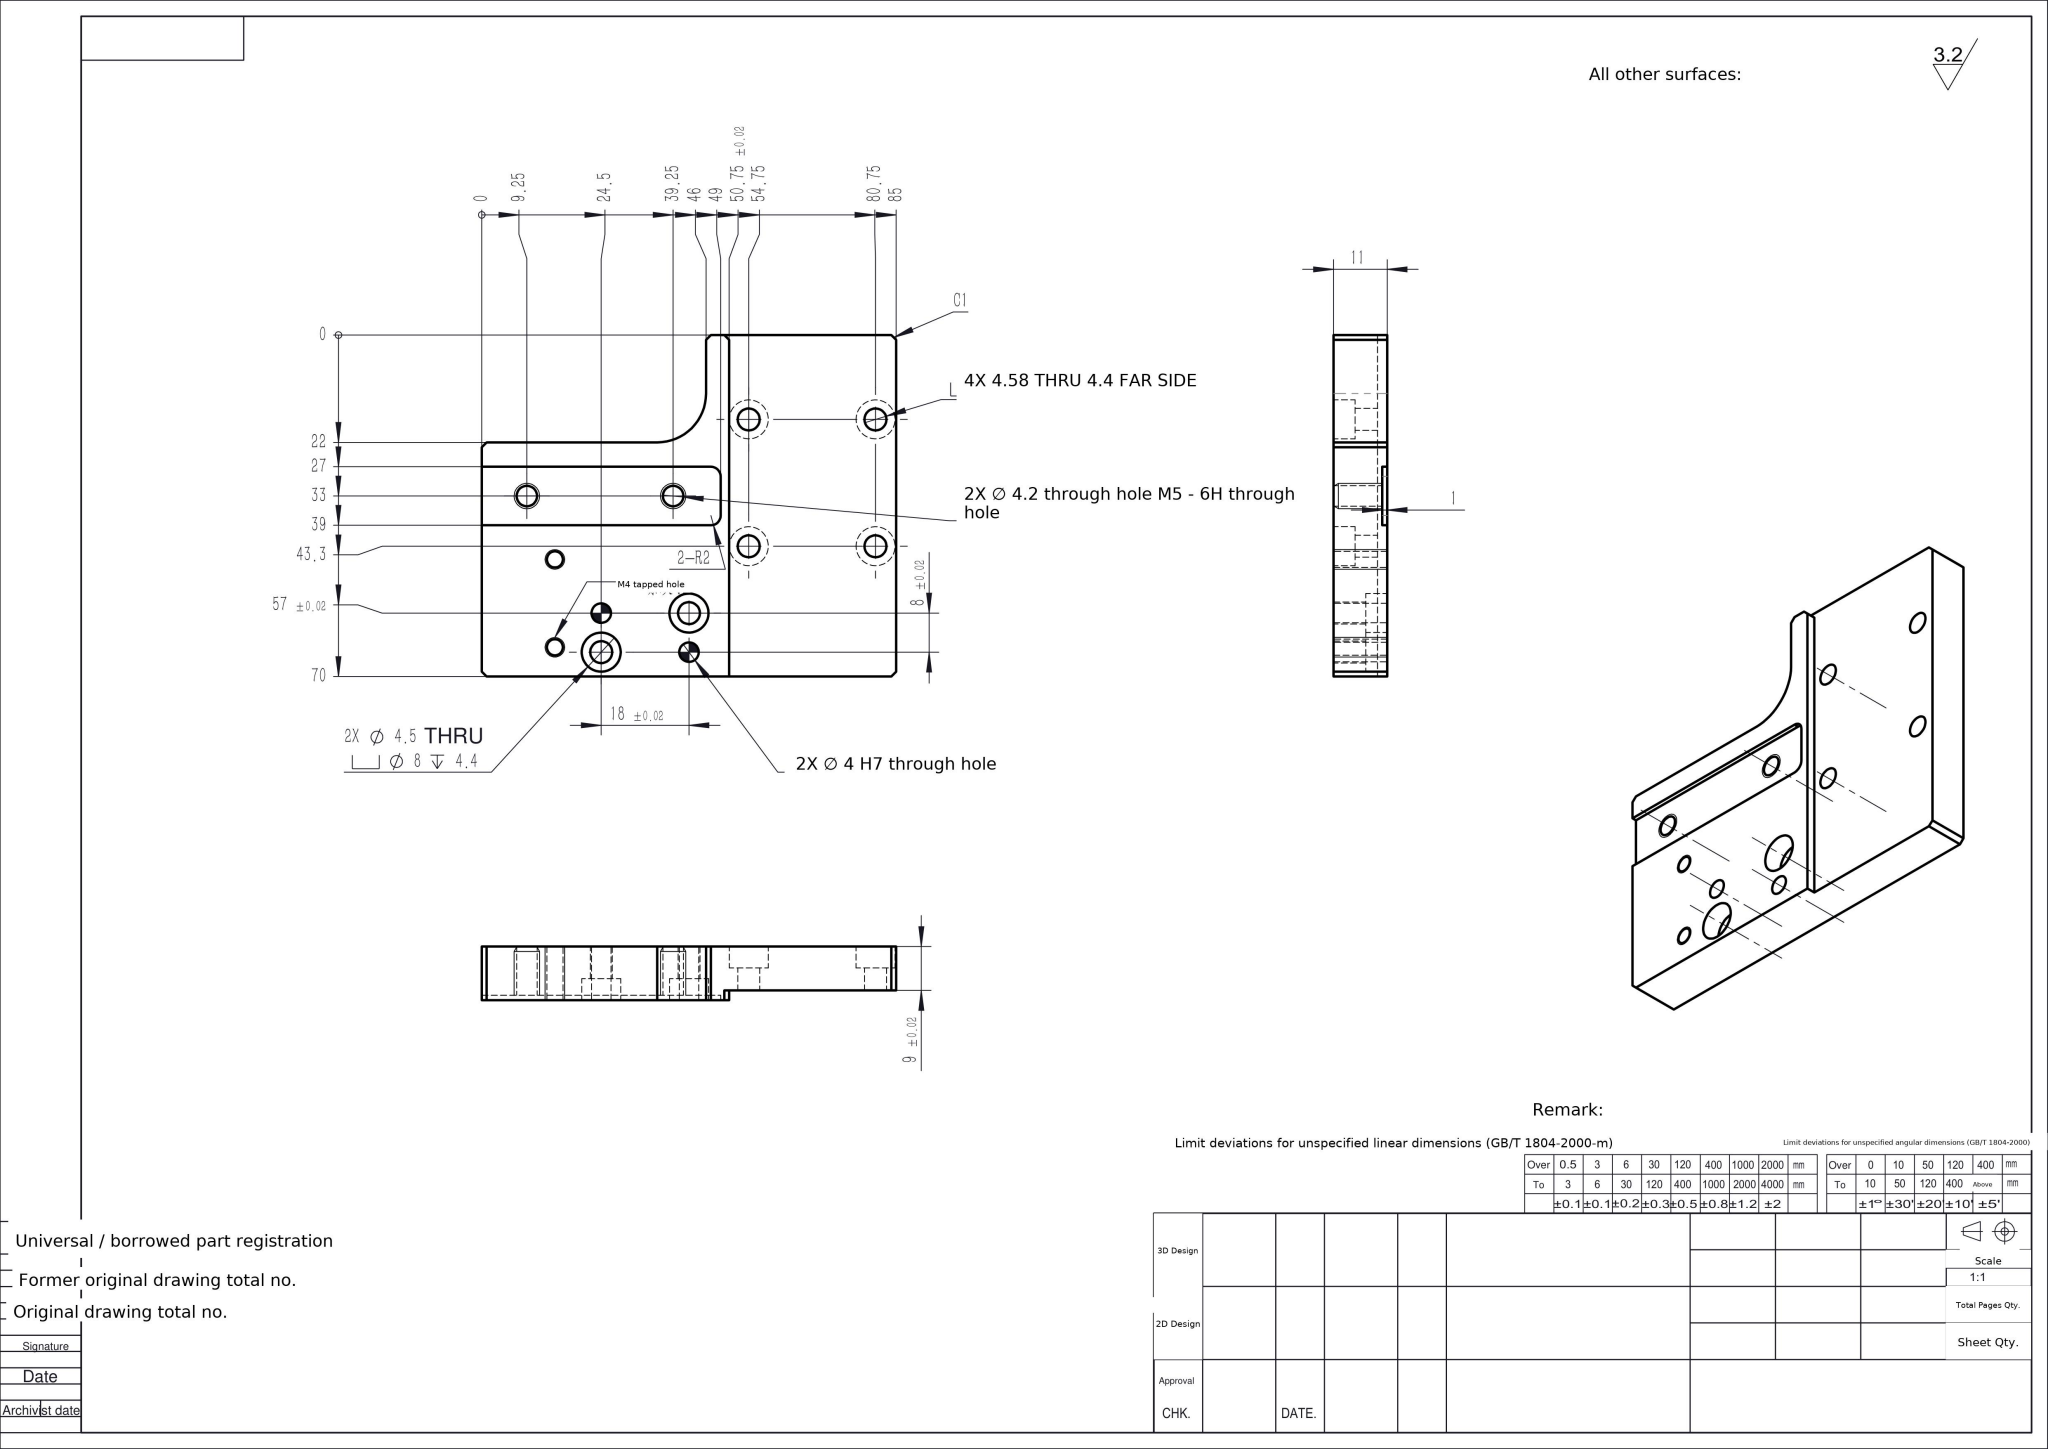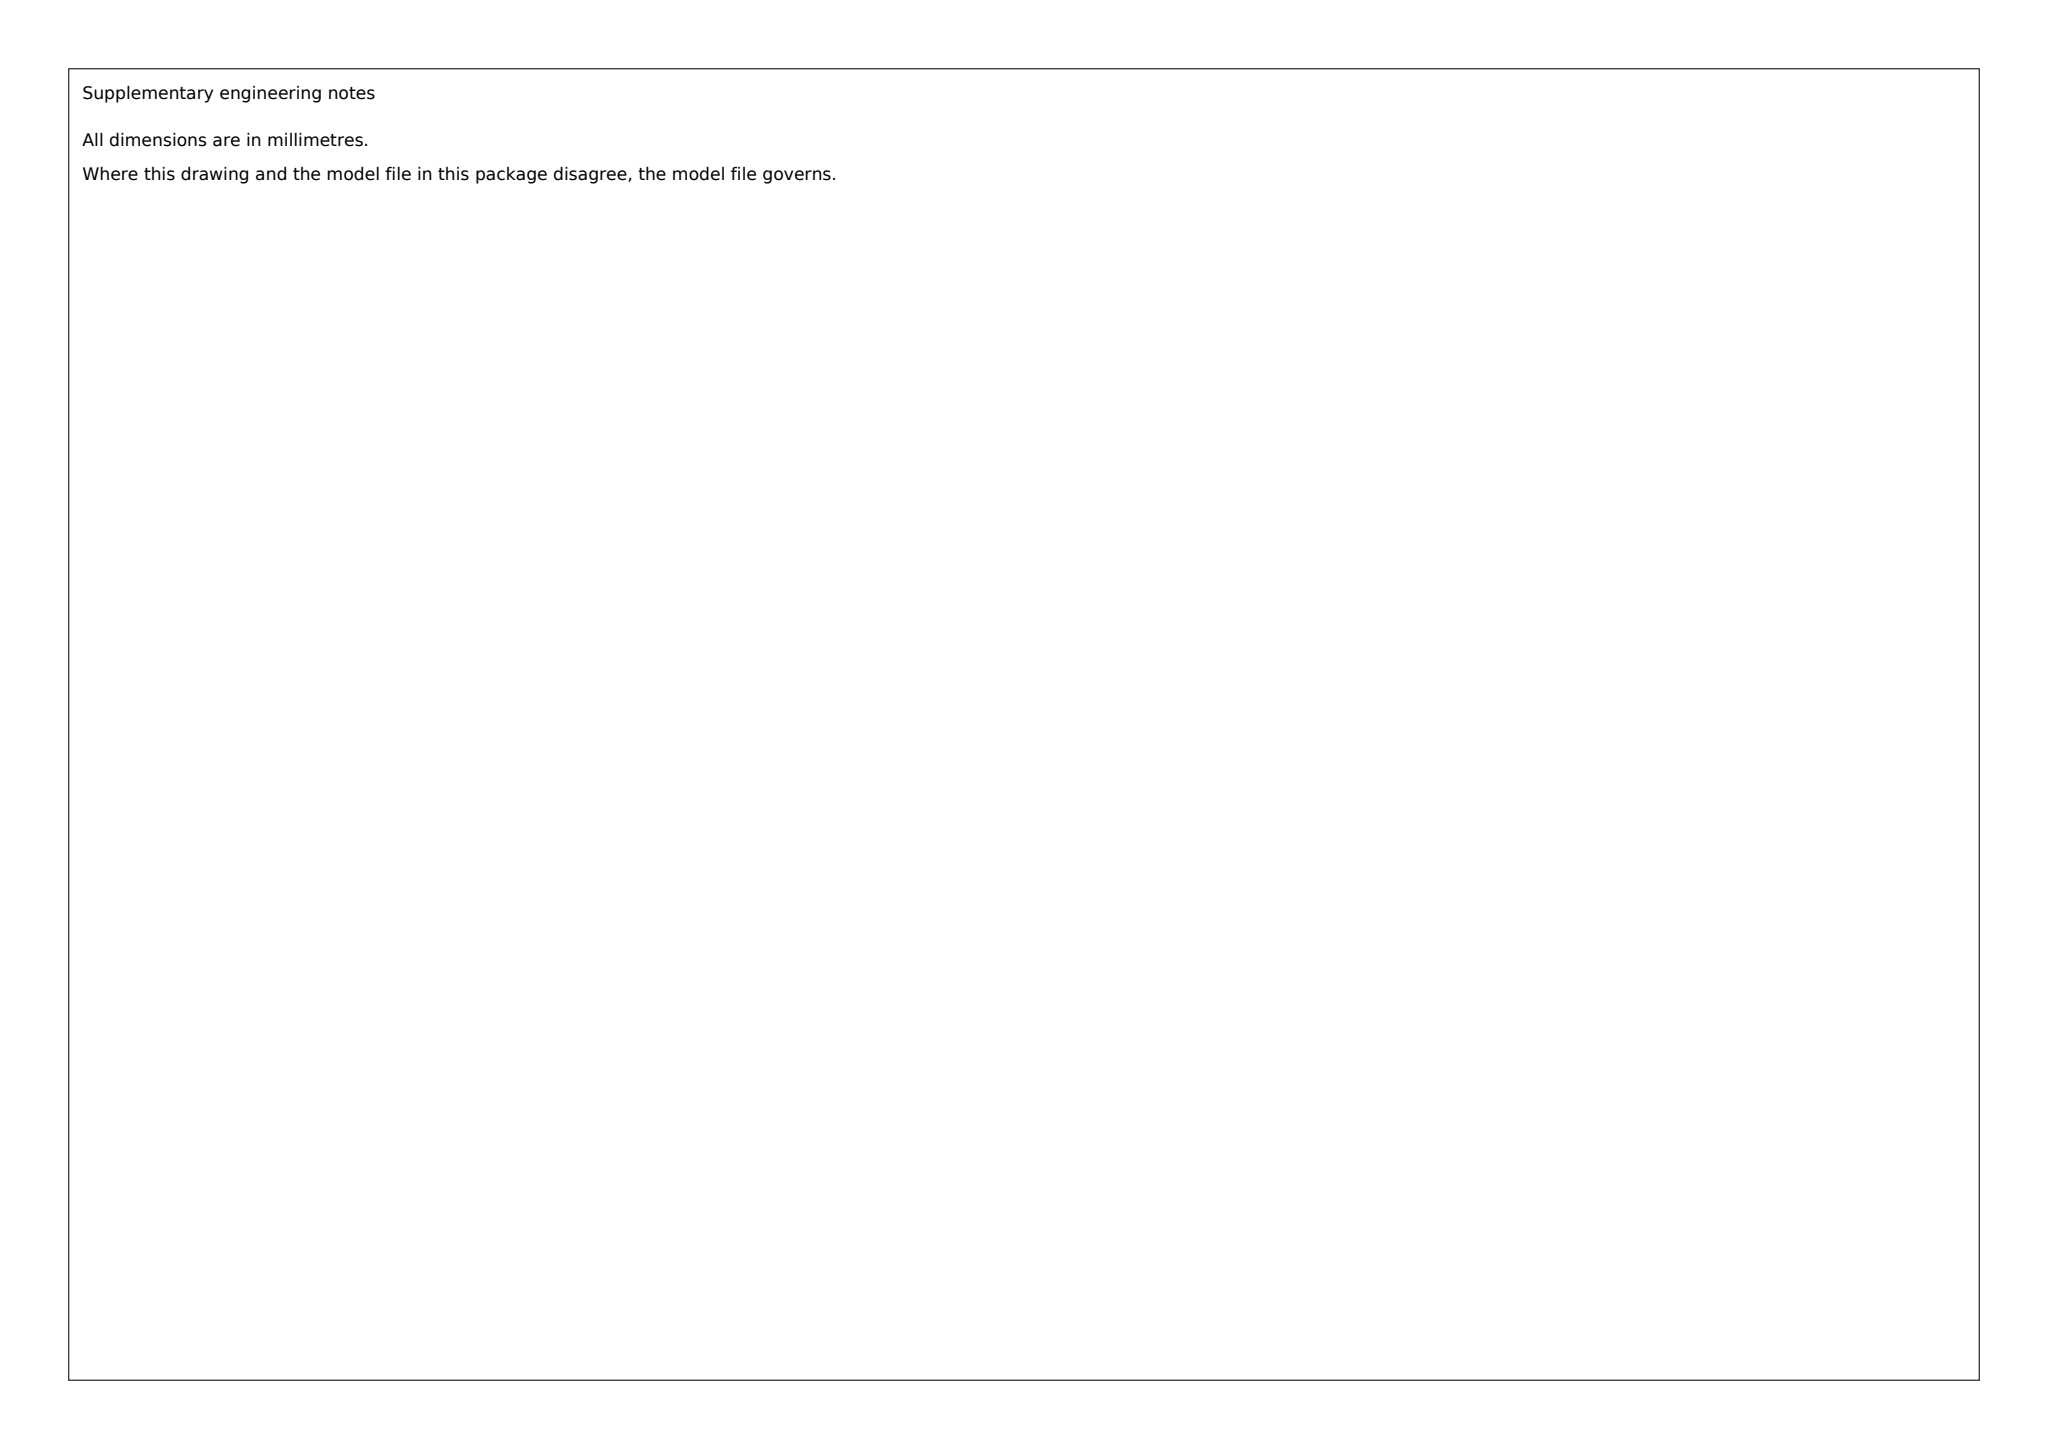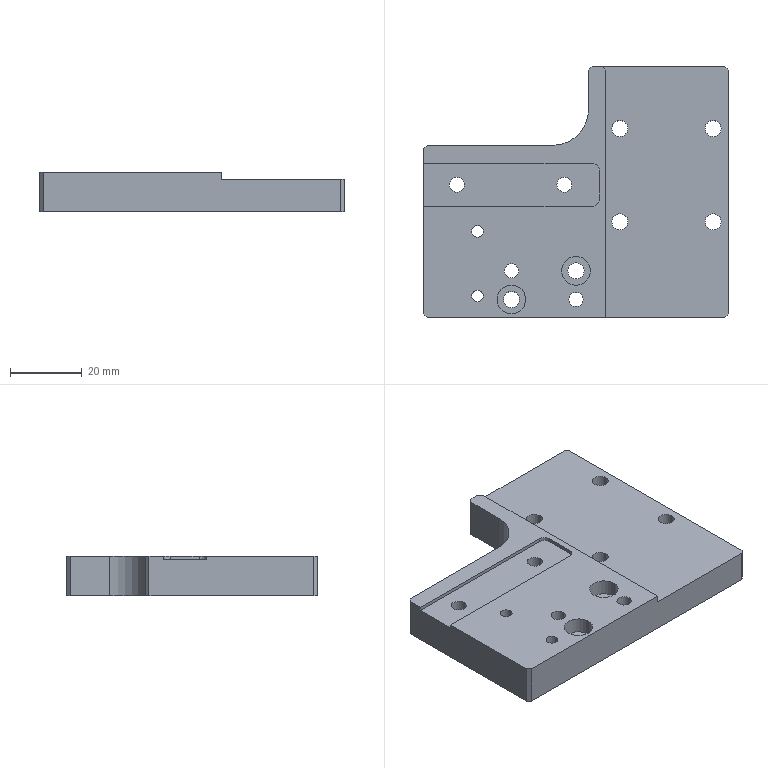Part | SolidWorks | mm | 1 solid | 65 faces | box 85 x 70 x 11 mm | volume 46575 mm3 | cylinder 39 | plane 26 | commonest cylinder face diameters 8 x12 4.5 x12 4 x6 3.3 x4 4.2 x4 20 x1
build123d program:
from build123d import *

# Parameters (mm, degrees)
SKETCH1_W                                       = 85
SKETCH1_H                                       = 70
BOSS_EXTRUDE1_DEPTH                             = 11
CUT_EXTRUDE1_DEPTH                              = 57.145
CUT_EXTRUDE1_DEPTH_BACK                         = 57.145
SKETCH3_W                                       = 46
SKETCH3_H                                       = 22
FILLET1_R                                       = 10
SKETCH4_W                                       = 50
SKETCH4_H                                       = 2
CUT_EXTRUDE2_DEPTH                              = 83.627
M4_HEX_SOCKET_HEAD_CAP_SCREW_CBORE2_D           = 4.5
M4_HEX_SOCKET_HEAD_CAP_SCREW_CBORE2_CBORE_D     = 8
M4_HEX_SOCKET_HEAD_CAP_SCREW_CBORE2_CBORE_DEPTH = 4.4
M5_TAPPED_HOLE2_D                               = 4.2
CHAMFER1_SIZE                                   = 1
SIZE_MM_DOWEL_PIN_HOLE_0_D                      = 4
M4_HEX_SOCKET_HEAD_CAP_SCREW_CBORE1_D           = 4.5
M4_HEX_SOCKET_HEAD_CAP_SCREW_CBORE1_CBORE_D     = 8
M4_HEX_SOCKET_HEAD_CAP_SCREW_CBORE1_CBORE_DEPTH = 4.4
SKETCH13_W                                      = 55
SKETCH13_H                                      = 12
CUT_EXTRUDE3_DEPTH                              = 1
FILLET2_R                                       = 2
M4_TAPPED_HOLE1_D                               = 3.3
M4_TAPPED_HOLE1_DEPTH                           = 14.1
M4_TAPPED_HOLE1_TIP                             = 0.9914


with BuildPart() as part:
    # Sketch1 → Boss-Extrude1 (new body)
    with BuildSketch(Plane.XY):
        Rectangle(SKETCH1_W, SKETCH1_H)
    extrude(amount=BOSS_EXTRUDE1_DEPTH)

    # Sketch3 → Cut-Extrude1 (cut, two sides: drawn at the far end of the back side and taken through both)
    with BuildSketch(Plane.XY.offset(11).offset(-CUT_EXTRUDE1_DEPTH_BACK)):
        with Locations((-19.5, 24)):
            Rectangle(SKETCH3_W, SKETCH3_H)
    extrude(amount=CUT_EXTRUDE1_DEPTH + CUT_EXTRUDE1_DEPTH_BACK, mode=Mode.SUBTRACT)

    # Fillet1
    fillet1_edges = [part.edges().sort_by_distance(p)[0] for p in [
        (3.5, 13, 5.5),
    ]]
    fillet(fillet1_edges, radius=FILLET1_R)

    # Sketch4 → Cut-Extrude2 (cut, through all)
    with BuildSketch(Plane(origin=(0, 35, 0), x_dir=(1, 0, 0), z_dir=(0, 1, 0))):
        with Locations((33.25, -10)):
            Rectangle(SKETCH4_W, SKETCH4_H)
    extrude(amount=-CUT_EXTRUDE2_DEPTH, mode=Mode.SUBTRACT)

    # M4 Hex Socket Head Cap Screw CBORE2 (through all)
    with Locations(Plane(origin=(0, 0, 0), x_dir=(1, 0, 0), z_dir=(0, 0, -1))):
        with Locations((12.25, -17.7), (12.25, 8.3), (38.25, 8.3), (38.25, -17.7)):
            CounterBoreHole(M4_HEX_SOCKET_HEAD_CAP_SCREW_CBORE2_D / 2, M4_HEX_SOCKET_HEAD_CAP_SCREW_CBORE2_CBORE_D / 2, M4_HEX_SOCKET_HEAD_CAP_SCREW_CBORE2_CBORE_DEPTH)

    # M5 Tapped Hole2 (through all)
    with Locations(Plane.XY.offset(11)):
        with Locations((-3.25, 2), (-33.25, 2)):
            Hole(M5_TAPPED_HOLE2_D / 2)

    # Chamfer1
    chamfer1_edges = [part.edges().sort_by_distance(p)[0] for p in [
        (-42.5, 13, 5.5),
        (3.5, 35, 5.5),
        (42.5, -35, 4.5),
        (42.5, 35, 4.5),
        (8.25, 35, 10),
        (-42.5, -35, 5.5),
    ]]
    chamfer(chamfer1_edges, length=CHAMFER1_SIZE)

    # Size mm Dowel Pin Hole 0 (through all)
    with Locations(Plane.XY.offset(11)):
        with Locations((-18, -22), (0, -30)):
            Hole(SIZE_MM_DOWEL_PIN_HOLE_0_D / 2)

    # M4 Hex Socket Head Cap Screw CBORE1 (through all)
    with Locations(Plane.XY.offset(11)):
        with Locations((-18, -30), (0, -22)):
            CounterBoreHole(M4_HEX_SOCKET_HEAD_CAP_SCREW_CBORE1_D / 2, M4_HEX_SOCKET_HEAD_CAP_SCREW_CBORE1_CBORE_D / 2, M4_HEX_SOCKET_HEAD_CAP_SCREW_CBORE1_CBORE_DEPTH)

    # Sketch13 → Cut-Extrude3 (cut)
    with BuildSketch(Plane.XY.offset(11)):
        with Locations((-21, 2)):
            Rectangle(SKETCH13_W, SKETCH13_H)
    extrude(amount=-CUT_EXTRUDE3_DEPTH, mode=Mode.SUBTRACT)

    # Fillet2
    fillet2_edges = [part.edges().sort_by_distance(p)[0] for p in [
        (6.5, -4, 10.5),
        (6.5, 8, 10.5),
    ]]
    fillet(fillet2_edges, radius=FILLET2_R)

    # M4 Tapped Hole1
    with Locations(Plane.XY.offset(11)):
        with Locations((-27.5, -11), (-27.5, -29)):
            Hole(M4_TAPPED_HOLE1_D / 2, depth=M4_TAPPED_HOLE1_DEPTH)
            with Locations((0, 0, -(M4_TAPPED_HOLE1_DEPTH + M4_TAPPED_HOLE1_TIP / 2))):  # 118° drill point
                Cone(0, M4_TAPPED_HOLE1_D / 2, M4_TAPPED_HOLE1_TIP, mode=Mode.SUBTRACT)


solid = part.part